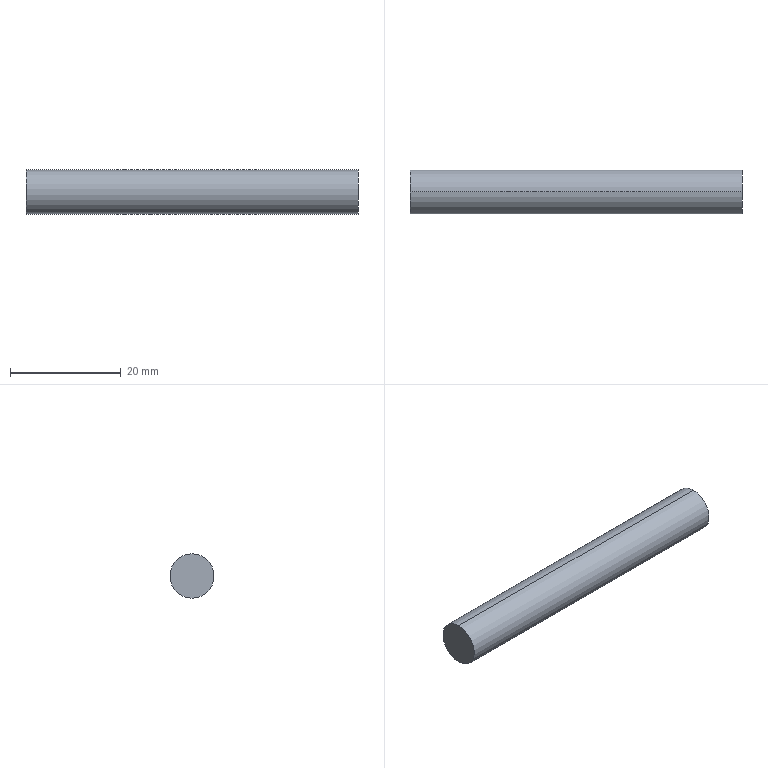Component | SolidWorks | DoubleFilmTransport-1_LimitAdjustmentScrew-1 | 1 solid | 4 faces | box 60 x 8 x 8 mm | volume 3016 mm3 | cylinder 2 | plane 2 | commonest cylinder face diameters 8 x2
build123d program:
from build123d import *

# Parameters (mm, degrees)
SKETCH1_W = 4
SKETCH1_H = 60


with BuildPart() as part:
    # Sketch1 → Revolve1 (revolve)
    with BuildSketch(Plane.XZ, mode=Mode.PRIVATE) as revolve1_sk:
        with Locations((2, 0)):
            Rectangle(SKETCH1_W, SKETCH1_H)
    revolve(revolve1_sk.sketch.rotate(Axis((0, 0, 30), (0, 0, -1)), 180), axis=Axis((0, 0, 30), (0, 0, -1)))


solid = part.part

# Placed as in the assembly
solid = solid.moved(Location((-296.246, 165.373, 13.5), (0, 90, 0)))
STEP:
#1=COLOUR_RGB('',0.7922,0.8196,0.9333);
#2=FILL_AREA_STYLE_COLOUR('',#1);
#3=FILL_AREA_STYLE('',(#2));
#4=SURFACE_STYLE_FILL_AREA(#3);
#5=SURFACE_SIDE_STYLE('',(#4));
#6=SURFACE_STYLE_USAGE(.BOTH.,#5);
#7=PRESENTATION_STYLE_ASSIGNMENT((#6));
#8=CARTESIAN_POINT('',(-12.844,6.511,0.374));
#9=VERTEX_POINT('',#8);
#10=CARTESIAN_POINT('',(-12.844,6.511,0.689));
#11=VERTEX_POINT('',#10);
#12=CARTESIAN_POINT('',(-12.844,6.511,0.5315));
#13=DIRECTION('',(1.,0.,0.));
#14=DIRECTION('',(0.,0.,-1.));
#15=AXIS2_PLACEMENT_3D('',#12,#13,#14);
#16=CIRCLE('',#15,0.1575);
#17=EDGE_CURVE('',#9,#11,#16,.T.);
#18=ORIENTED_EDGE('',*,*,#17,.T.);
#19=CARTESIAN_POINT('',(-10.482,6.511,0.689));
#20=VERTEX_POINT('',#19);
#21=CARTESIAN_POINT('',(-12.844,6.511,0.689));
#22=DIRECTION('',(1.,0.,0.));
#23=VECTOR('',#22,39.37);
#24=LINE('',#21,#23);
#25=EDGE_CURVE('',#11,#20,#24,.T.);
#26=ORIENTED_EDGE('',*,*,#25,.T.);
#27=CARTESIAN_POINT('',(-10.482,6.511,0.374));
#28=VERTEX_POINT('',#27);
#29=CARTESIAN_POINT('',(-10.482,6.511,0.5315));
#30=DIRECTION('',(1.,0.,0.));
#31=DIRECTION('',(0.,0.,-1.));
#32=AXIS2_PLACEMENT_3D('',#29,#30,#31);
#33=CIRCLE('',#32,0.1575);
#34=EDGE_CURVE('',#28,#20,#33,.T.);
#35=ORIENTED_EDGE('',*,*,#34,.F.);
#36=CARTESIAN_POINT('',(-12.844,6.511,0.374));
#37=DIRECTION('',(1.,0.,0.));
#38=VECTOR('',#37,39.37);
#39=LINE('',#36,#38);
#40=EDGE_CURVE('',#9,#28,#39,.T.);
#41=ORIENTED_EDGE('',*,*,#40,.F.);
#42=EDGE_LOOP('',(#18,#26,#35,#41));
#43=FACE_OUTER_BOUND('',#42,.T.);
#44=CARTESIAN_POINT('',(-12.844,6.511,0.5315));
#45=DIRECTION('',(1.,0.,0.));
#46=DIRECTION('',(0.,0.,-1.));
#47=AXIS2_PLACEMENT_3D('',#44,#45,#46);
#48=CYLINDRICAL_SURFACE('',#47,0.1575);
#49=ADVANCED_FACE('',(#43),#48,.T.);
#50=ORIENTED_EDGE('',*,*,#25,.F.);
#51=CARTESIAN_POINT('',(-12.844,6.511,0.5315));
#52=DIRECTION('',(1.,0.,0.));
#53=DIRECTION('',(0.,0.,-1.));
#54=AXIS2_PLACEMENT_3D('',#51,#52,#53);
#55=CIRCLE('',#54,0.1575);
#56=EDGE_CURVE('',#11,#9,#55,.T.);
#57=ORIENTED_EDGE('',*,*,#56,.T.);
#58=ORIENTED_EDGE('',*,*,#40,.T.);
#59=CARTESIAN_POINT('',(-10.482,6.511,0.5315));
#60=DIRECTION('',(1.,0.,0.));
#61=DIRECTION('',(0.,0.,-1.));
#62=AXIS2_PLACEMENT_3D('',#59,#60,#61);
#63=CIRCLE('',#62,0.1575);
#64=EDGE_CURVE('',#20,#28,#63,.T.);
#65=ORIENTED_EDGE('',*,*,#64,.F.);
#66=EDGE_LOOP('',(#50,#57,#58,#65));
#67=FACE_OUTER_BOUND('',#66,.T.);
#68=CARTESIAN_POINT('',(-12.844,6.511,0.5315));
#69=DIRECTION('',(1.,0.,0.));
#70=DIRECTION('',(0.,0.,-1.));
#71=AXIS2_PLACEMENT_3D('',#68,#69,#70);
#72=CYLINDRICAL_SURFACE('',#71,0.1575);
#73=ADVANCED_FACE('',(#67),#72,.T.);
#74=ORIENTED_EDGE('',*,*,#17,.F.);
#75=ORIENTED_EDGE('',*,*,#56,.F.);
#76=EDGE_LOOP('',(#74,#75));
#77=FACE_OUTER_BOUND('',#76,.T.);
#78=CARTESIAN_POINT('',(-12.844,6.511,0.689));
#79=DIRECTION('',(-1.,0.,0.));
#80=DIRECTION('',(0.,0.,1.));
#81=AXIS2_PLACEMENT_3D('',#78,#79,#80);
#82=PLANE('',#81);
#83=ADVANCED_FACE('',(#77),#82,.T.);
#84=ORIENTED_EDGE('',*,*,#34,.T.);
#85=ORIENTED_EDGE('',*,*,#64,.T.);
#86=EDGE_LOOP('',(#84,#85));
#87=FACE_OUTER_BOUND('',#86,.T.);
#88=CARTESIAN_POINT('',(-10.482,6.511,0.5315));
#89=DIRECTION('',(1.,0.,0.));
#90=DIRECTION('',(0.,0.,-1.));
#91=AXIS2_PLACEMENT_3D('',#88,#89,#90);
#92=PLANE('',#91);
#93=ADVANCED_FACE('',(#87),#92,.T.);
#94=CLOSED_SHELL('',(#49,#73,#83,#93));
#95=MANIFOLD_SOLID_BREP('',#94);
#96=STYLED_ITEM('',(#7),#95);
#97=PRESENTATION_LAYER_ASSIGNMENT('','',(#96));
#98=CARTESIAN_POINT('',(0.,0.,0.));
#99=DIRECTION('',(0.,0.,1.));
#100=DIRECTION('',(1.,0.,0.));
#101=AXIS2_PLACEMENT_3D('',#98,#99,#100);
#102=(LENGTH_UNIT()NAMED_UNIT(*)SI_UNIT($,.METRE.));
#103=LENGTH_MEASURE_WITH_UNIT(LENGTH_MEASURE(0.0254),#102);
#104=DIMENSIONAL_EXPONENTS(1.,0.,0.,0.,0.,0.,0.);
#105=(CONVERSION_BASED_UNIT('',#103)LENGTH_UNIT()NAMED_UNIT(#104));
#106=UNCERTAINTY_MEASURE_WITH_UNIT(LENGTH_MEASURE(0.00001),#105,'','');
#107=(NAMED_UNIT(*)PLANE_ANGLE_UNIT()SI_UNIT($,.RADIAN.));
#108=(NAMED_UNIT(*)SI_UNIT($,.STERADIAN.)SOLID_ANGLE_UNIT());
#109=(GEOMETRIC_REPRESENTATION_CONTEXT(3)GLOBAL_UNCERTAINTY_ASSIGNED_CONTEXT((#106))GLOBAL_UNIT_ASSIGNED_CONTEXT((#105,#107,#108))REPRESENTATION_CONTEXT('',''));
#110=ADVANCED_BREP_SHAPE_REPRESENTATION('',(#95,#101),#109);
#111=(LENGTH_UNIT()NAMED_UNIT(*)SI_UNIT($,.METRE.));
#112=LENGTH_MEASURE_WITH_UNIT(LENGTH_MEASURE(0.0254),#111);
#113=DIMENSIONAL_EXPONENTS(1.,0.,0.,0.,0.,0.,0.);
#114=(CONVERSION_BASED_UNIT('',#112)LENGTH_UNIT()NAMED_UNIT(#113));
#115=UNCERTAINTY_MEASURE_WITH_UNIT(LENGTH_MEASURE(0.00001),#114,'','');
#116=(NAMED_UNIT(*)PLANE_ANGLE_UNIT()SI_UNIT($,.RADIAN.));
#117=(NAMED_UNIT(*)SI_UNIT($,.STERADIAN.)SOLID_ANGLE_UNIT());
#118=(GEOMETRIC_REPRESENTATION_CONTEXT(3)GLOBAL_UNCERTAINTY_ASSIGNED_CONTEXT((#115))GLOBAL_UNIT_ASSIGNED_CONTEXT((#114,#116,#117))REPRESENTATION_CONTEXT('',''));
#119=MECHANICAL_DESIGN_GEOMETRIC_PRESENTATION_REPRESENTATION('',(#96),#118);